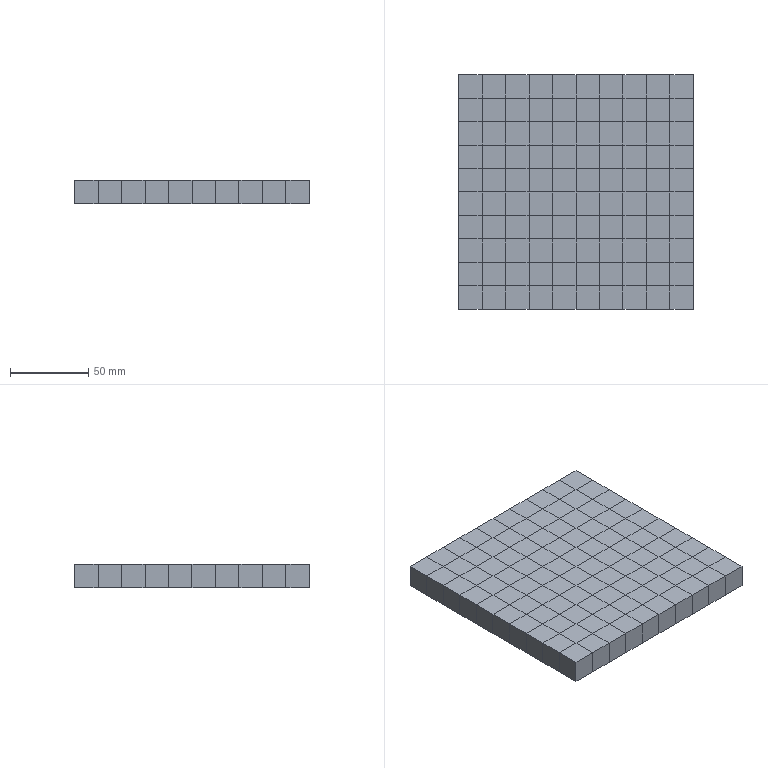Component | NX | 10_WORKPIECE | 100 solids | 600 faces | volume 337500 mm3 | plane 600